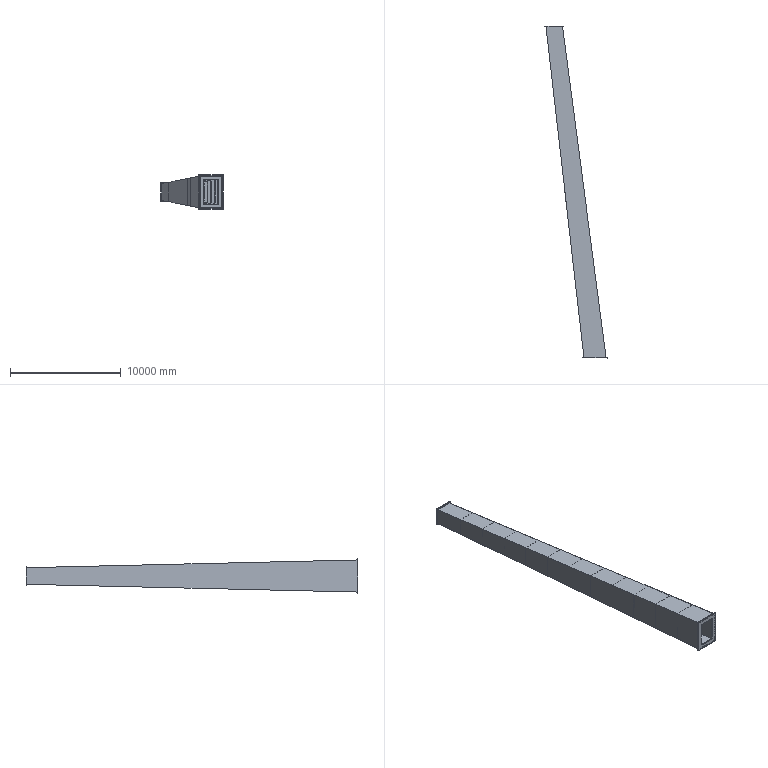Component | SolidWorks | RigidLeg-1 | 1 solid | 257 faces | volume 11318303825 mm3 | cylinder 142 | plane 89 | spline 26 | commonest cylinder face diameters 40 x140 200 x2